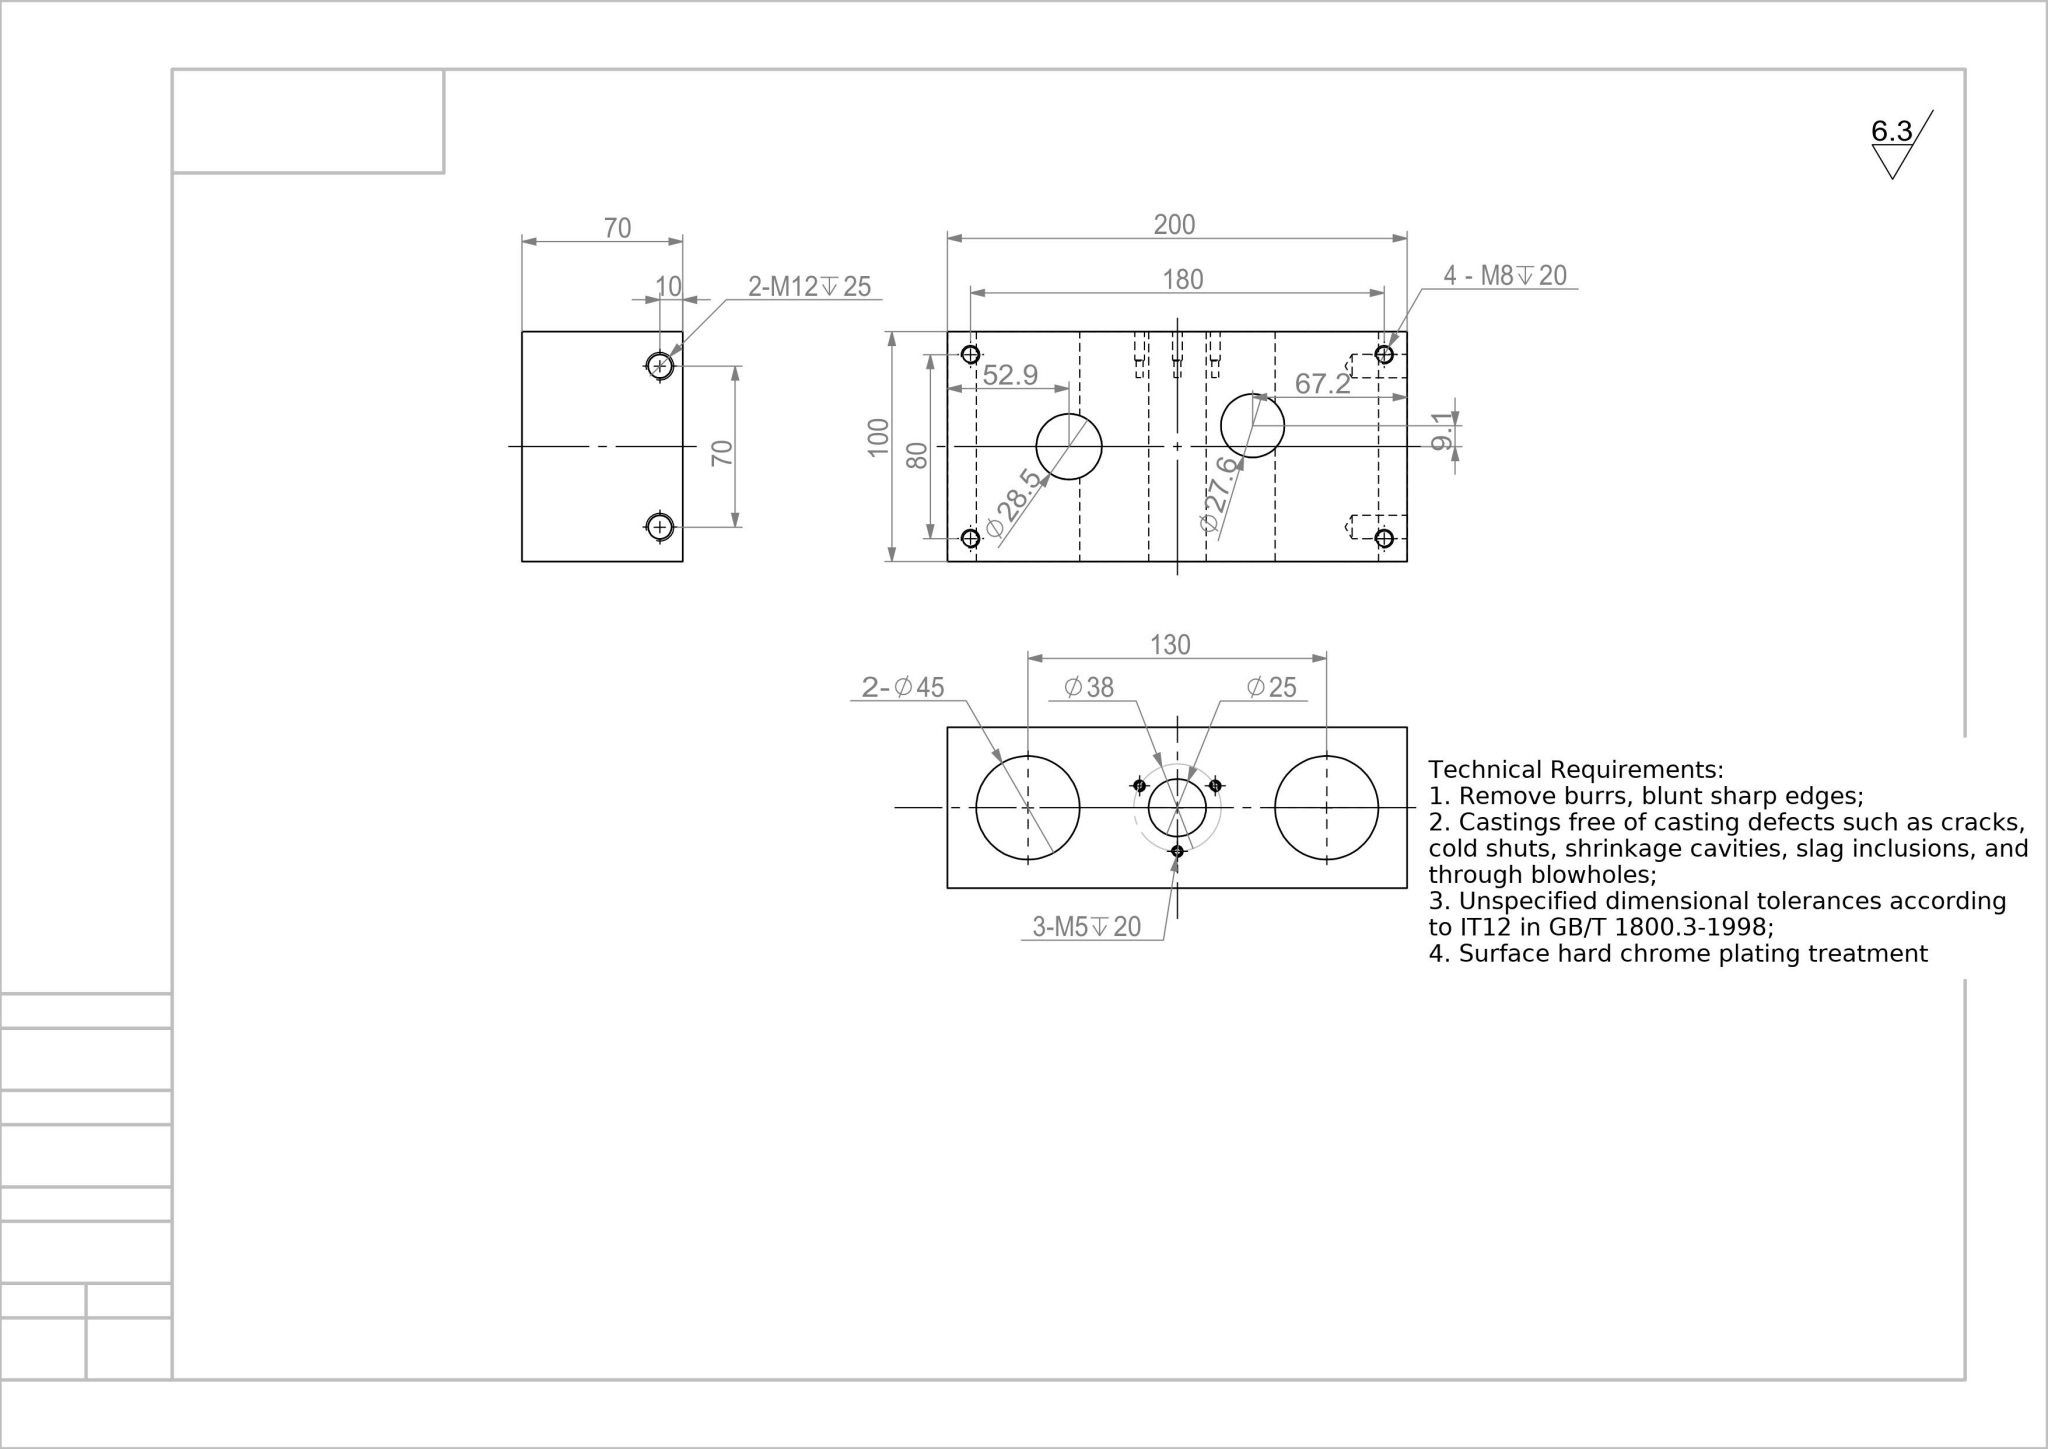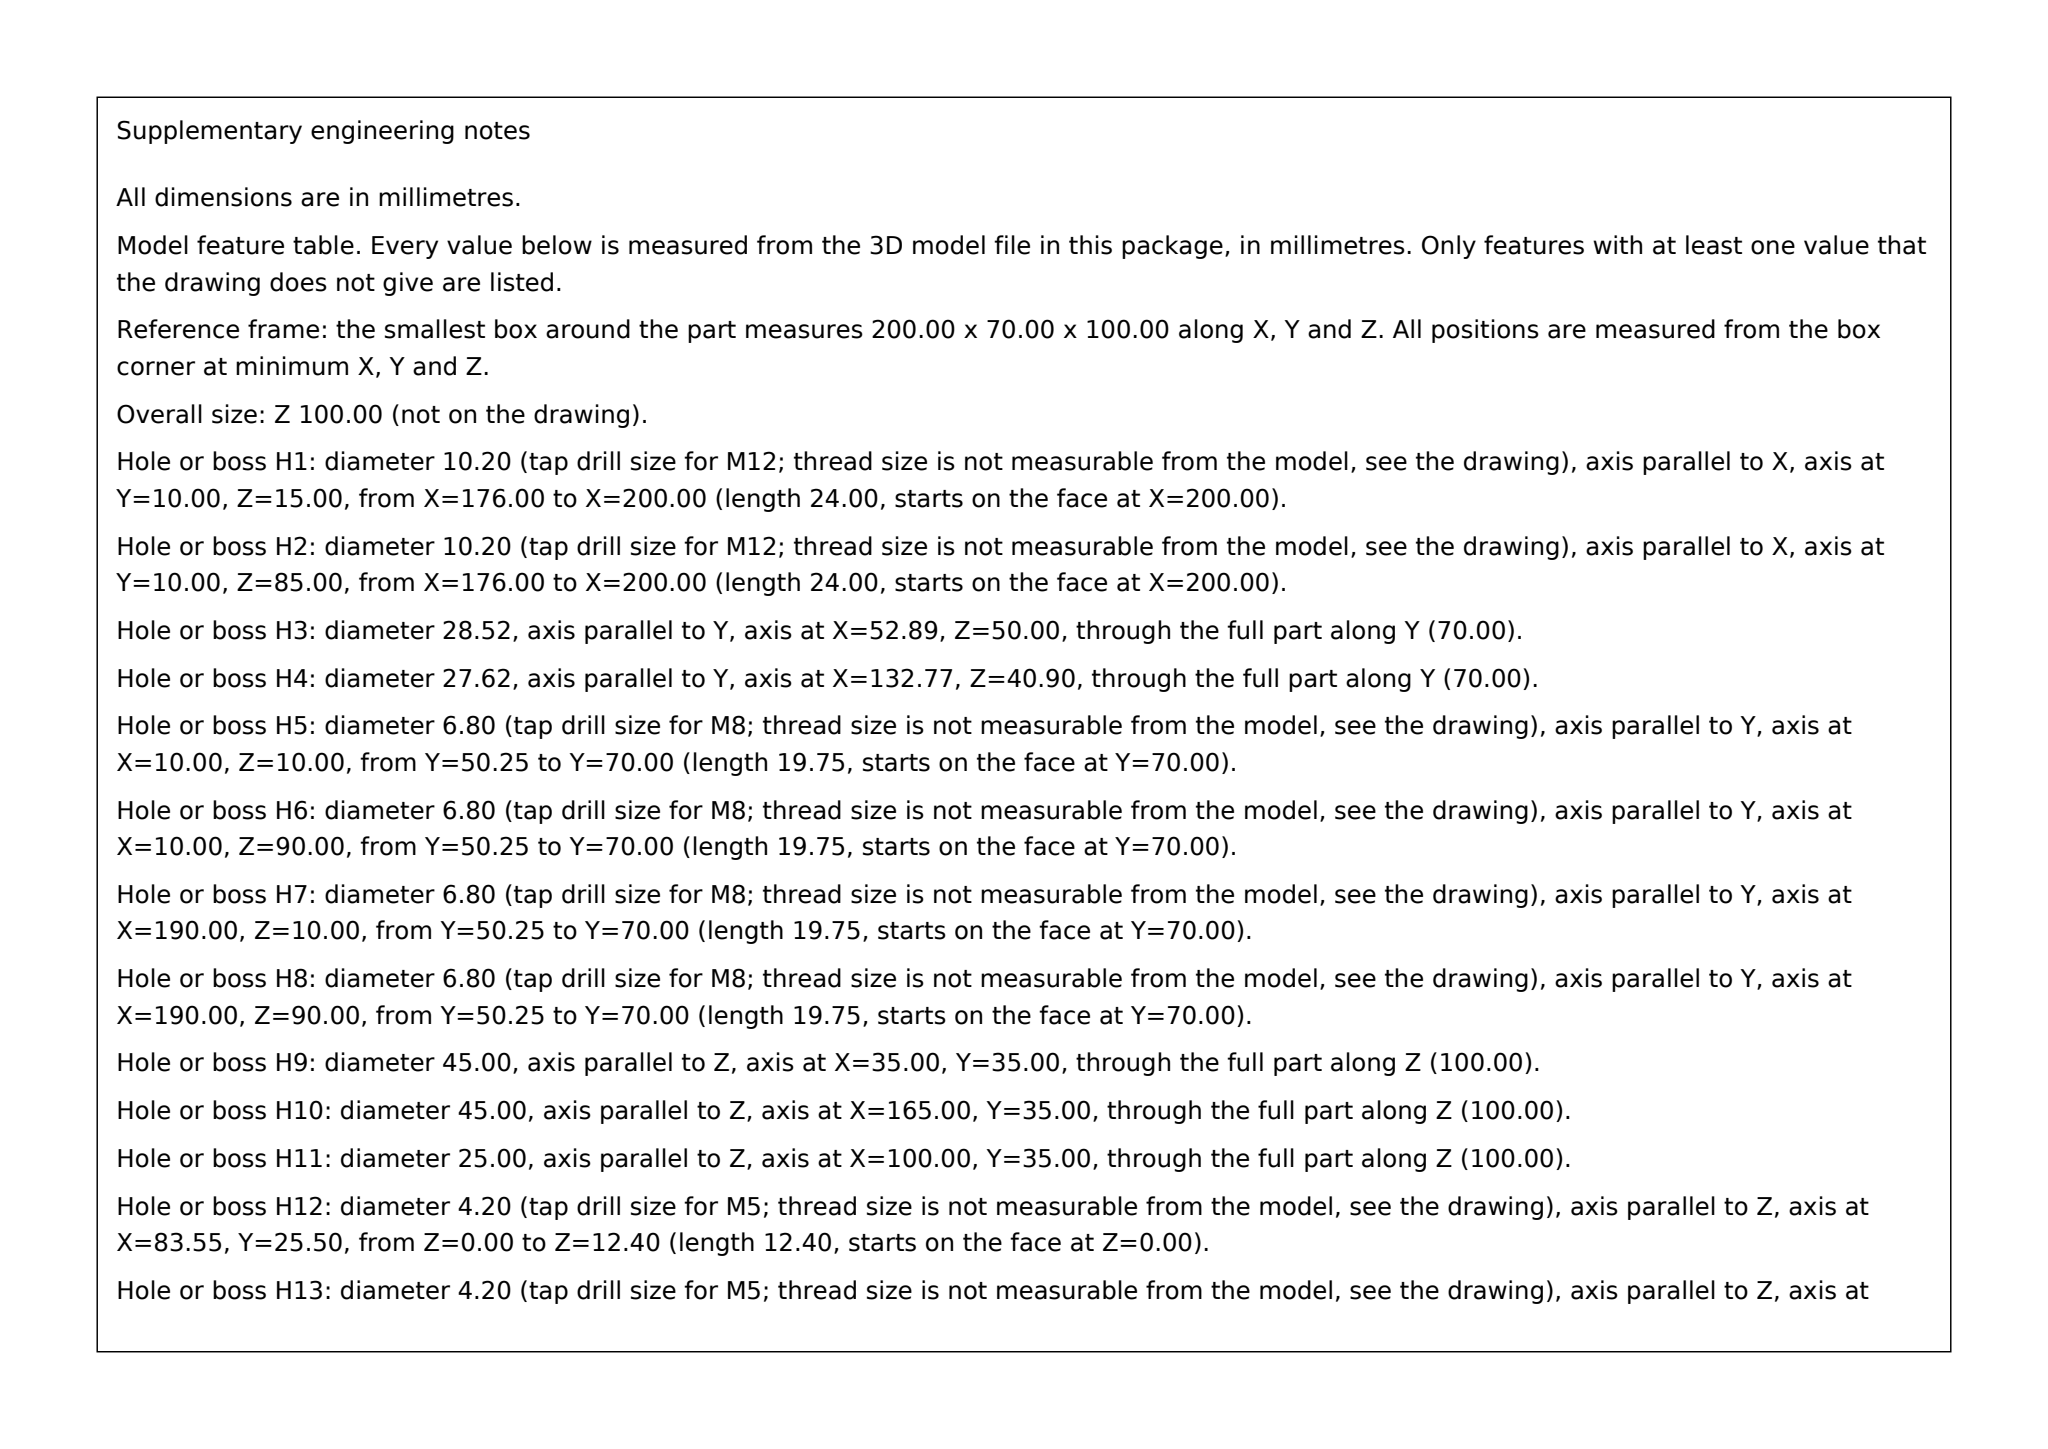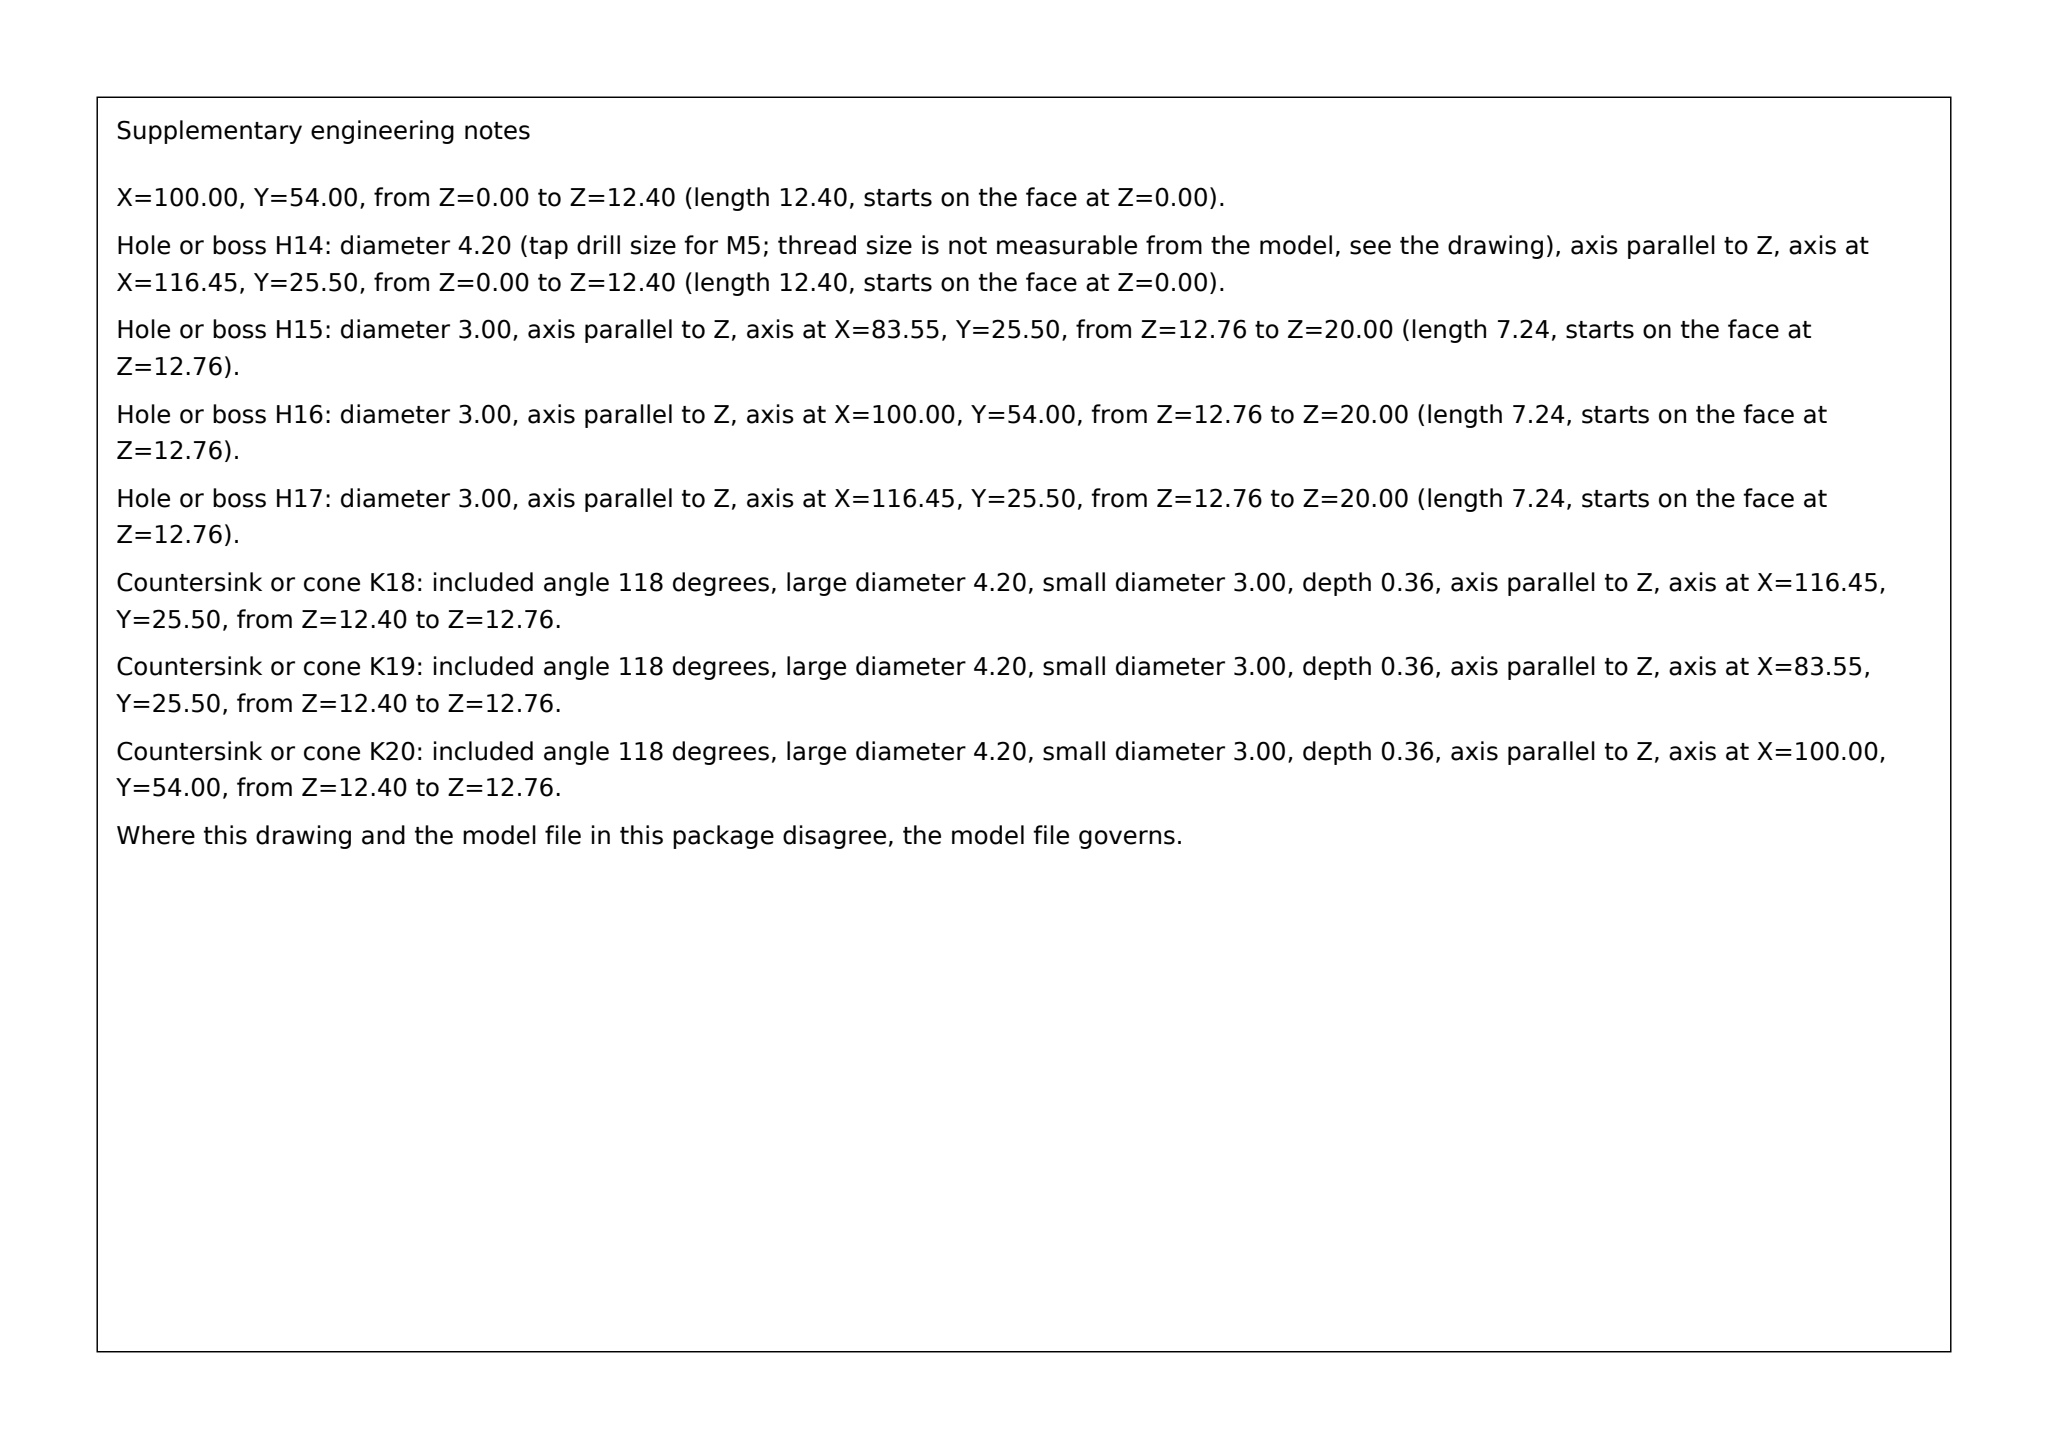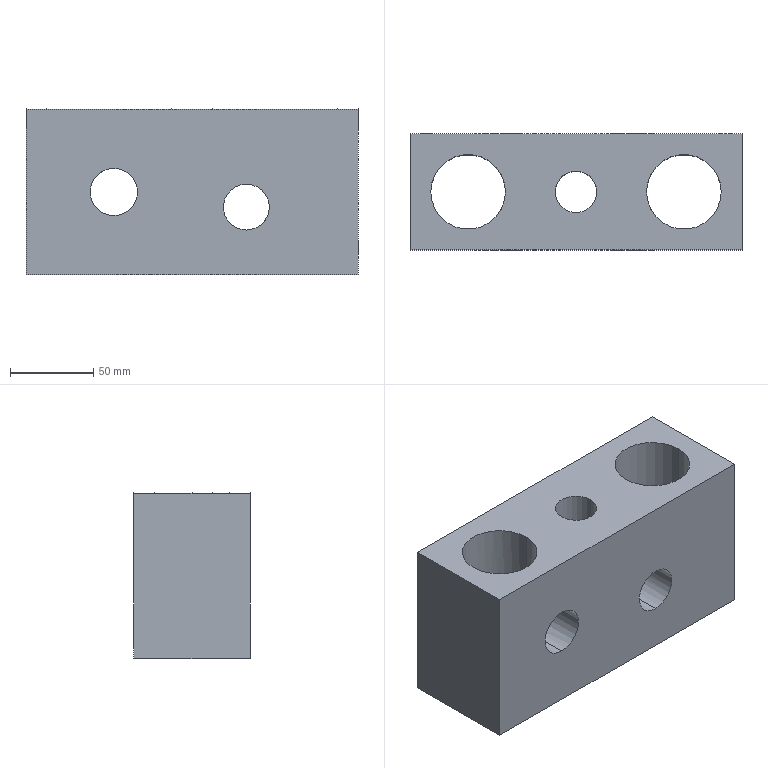Part | SolidWorks | mm | 1 solid | 62 faces | box 200 x 70 x 100 mm | volume 953623 mm3 | cylinder 35 | cone 18 | plane 9 | commonest cylinder face diameters 6.8 x8 3 x6 4.2 x6 10.2 x4 45 x4 28.515 x3 27.615 x2 25 x2
build123d program:
from build123d import *

# Parameters (mm, degrees)
SKETCH1_W              = 200
SKETCH1_H              = 70
SKETCH1_R              = 22.5
BOSS_EXTRUDE1_DEPTH    = 50
SKETCH2_R              = 12.5
CUT_EXTRUDE1_DEPTH     = 100
M12_TAPPED_HOLE1_D     = 10.2
M12_TAPPED_HOLE1_DEPTH = 24
M12_TAPPED_HOLE1_TIP   = 3.064
M8_TAPPED_HOLE1_D      = 6.8
M8_TAPPED_HOLE1_DEPTH  = 19.75
M8_TAPPED_HOLE1_TIP    = 2.043
SKETCH5_R              = 1.5
CUT_EXTRUDE2_DEPTH     = 20
M5_TAPPED_HOLE1_D      = 4.2
M5_TAPPED_HOLE1_DEPTH  = 12.4
M5_TAPPED_HOLE1_TIP    = 1.262
SKETCH7_R              = 14.258
SKETCH7_R_2            = 13.807
CUT_EXTRUDE3_DEPTH     = 80


with BuildPart() as part:
    # Sketch1 → Boss-Extrude1 (new, symmetric)
    with BuildSketch(Plane.XY):
        Rectangle(SKETCH1_W, SKETCH1_H)
        with Locations(Location((-65, 0, 0), (0, 0, 180))):
            Circle(SKETCH1_R, mode=Mode.SUBTRACT)
        with Locations(Location((65, 0, 0), (0, 0, 180))):
            Circle(SKETCH1_R, mode=Mode.SUBTRACT)
    extrude(amount=BOSS_EXTRUDE1_DEPTH, both=True)

    # Sketch2 → Cut-Extrude1 (cut)
    with BuildSketch(Plane.XY.offset(50)):
        Circle(SKETCH2_R)
    extrude(amount=-CUT_EXTRUDE1_DEPTH, mode=Mode.SUBTRACT)

    # M12 Tapped Hole1
    with Locations(Plane(origin=(100, -25, 35), x_dir=(0, 0, 1), z_dir=(1, 0, 0))):
        with Locations((0, 0), (-70, 0)):
            Hole(M12_TAPPED_HOLE1_D / 2, depth=M12_TAPPED_HOLE1_DEPTH)
            with Locations((0, 0, -(M12_TAPPED_HOLE1_DEPTH + M12_TAPPED_HOLE1_TIP / 2))):  # 118° drill point
                Cone(0, M12_TAPPED_HOLE1_D / 2, M12_TAPPED_HOLE1_TIP, mode=Mode.SUBTRACT)

    # M8 Tapped Hole1
    with Locations(Plane(origin=(90, 35, 40), x_dir=(0, 0, 1), z_dir=(0, 1, 0))):
        with Locations((0, 0), (0, -180), (-80, -180), (-80, 0)):
            Hole(M8_TAPPED_HOLE1_D / 2, depth=M8_TAPPED_HOLE1_DEPTH)
            with Locations((0, 0, -(M8_TAPPED_HOLE1_DEPTH + M8_TAPPED_HOLE1_TIP / 2))):  # 118° drill point
                Cone(0, M8_TAPPED_HOLE1_D / 2, M8_TAPPED_HOLE1_TIP, mode=Mode.SUBTRACT)

    # Sketch5 → Cut-Extrude2 (cut)
    with BuildSketch(Plane(origin=(0, 0, -50), x_dir=(-1, 0, 0), z_dir=(0, 0, -1))):
        with Locations((0, 19)):
            Circle(SKETCH5_R)
        with Locations((16.454, -9.5)):
            Circle(SKETCH5_R)
        with Locations((-16.454, -9.5)):
            Circle(SKETCH5_R)
    extrude(amount=-CUT_EXTRUDE2_DEPTH, mode=Mode.SUBTRACT)

    # M5 Tapped Hole1
    with Locations(Plane(origin=(16.454, -9.5, -50), x_dir=(-1, 0, 0), z_dir=(0, 0, -1))):
        with Locations((0, 0), (32.909, 0), (16.454, 28.5)):
            Hole(M5_TAPPED_HOLE1_D / 2, depth=M5_TAPPED_HOLE1_DEPTH)
            with Locations((0, 0, -(M5_TAPPED_HOLE1_DEPTH + M5_TAPPED_HOLE1_TIP / 2))):  # 118° drill point
                Cone(0, M5_TAPPED_HOLE1_D / 2, M5_TAPPED_HOLE1_TIP, mode=Mode.SUBTRACT)

    # Sketch7 → Cut-Extrude3 (cut)
    with BuildSketch(Plane(origin=(0, 35, 0), x_dir=(1, 0, 0), z_dir=(0, 1, 0))):
        with Locations(Location((-47.108, 0, 0), (0, 0, 270))):
            Circle(SKETCH7_R)
        with Locations(Location((32.771, 9.103, 0), (0, 0, 270))):
            Circle(SKETCH7_R_2)
    extrude(amount=-CUT_EXTRUDE3_DEPTH, mode=Mode.SUBTRACT)


solid = part.part